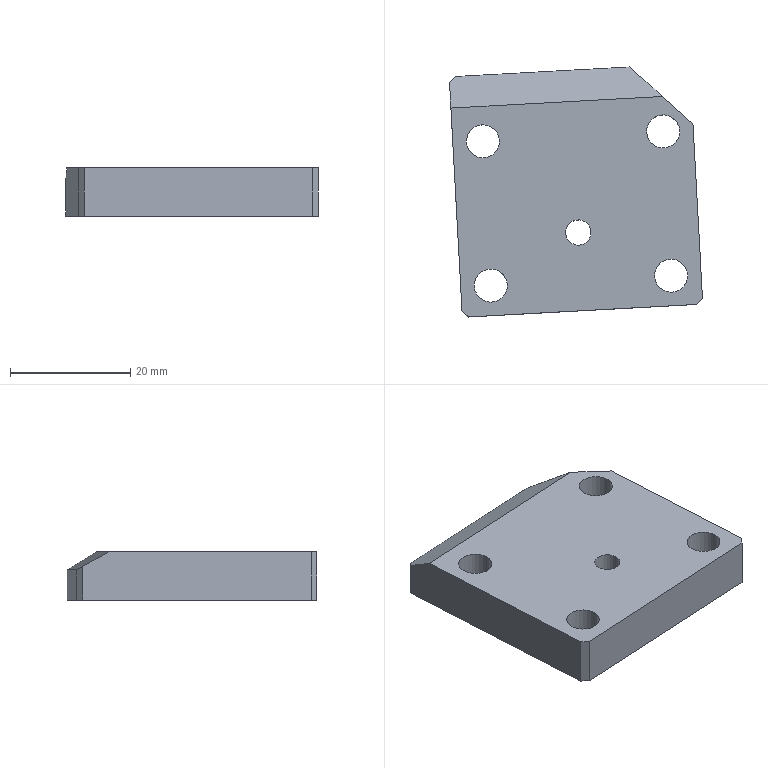Component | SolidWorks | T160418-M01U03-P11A-1 | 1 solid | 24 faces | box 42.02 x 41.53 x 8 mm | volume 10991 mm3 | cylinder 12 | plane 12 | commonest cylinder face diameters 5.5 x8 14 x2 4.2 x2 | material S45C
build123d program:
from build123d import *

# Parameters (mm, degrees)
SKETCH1_W            = 40
SKETCH1_H            = 40
BOSS_EXTRUDE1_DEPTH  = 8
M5_CLEARANCE_HOLE1_D = 5.5
M5_TAPPED_HOLE1_D    = 4.2
CHAMFER1_SIZE        = 10
CHAMFER2_SIZE        = 3
CHAMFER2_SIZE2       = 5.196
CHAMFER3_SIZE        = 1
SKETCH9_R            = 7
CUT_EXTRUDE3_DEPTH   = 2


with BuildPart() as part:
    # Sketch1 → Boss-Extrude1 (new body)
    with BuildSketch(Plane.XY):
        Rectangle(SKETCH1_W, SKETCH1_H)
    extrude(amount=BOSS_EXTRUDE1_DEPTH)

    # M5 Clearance Hole1 (through all)
    with Locations(Plane.XY.offset(8)):
        with Locations((-15, 9), (-15, -15), (15, -15), (15, 9)):
            Hole(M5_CLEARANCE_HOLE1_D / 2)

    # M5 Tapped Hole1 (through all)
    with Locations(Plane.XY.offset(8)):
        with Locations((0, -7)):
            Hole(M5_TAPPED_HOLE1_D / 2)

    # Chamfer1
    chamfer1_edges = [part.edges().sort_by_distance(p)[0] for p in [
        (-20, 20, 4),
    ]]
    chamfer(chamfer1_edges, length=CHAMFER1_SIZE)

    # Chamfer2
    chamfer2_edges = [part.edges().sort_by_distance(p)[0] for p in [
        (5, 20, 0),
    ]]
    chamfer2_side = [part.faces().sort_by_distance(p)[0] for p in [
        (5, 20, 4),
    ]]
    chamfer(chamfer2_edges, length=CHAMFER2_SIZE, length2=CHAMFER2_SIZE2, reference=chamfer2_side[0])

    # Chamfer3
    chamfer3_edges = [part.edges().sort_by_distance(p)[0] for p in [
        (20, -20, 4),
        (-20, -20, 4),
        (20, 20, 5.5),
    ]]
    chamfer(chamfer3_edges, length=CHAMFER3_SIZE)

    # Sketch9 → Cut-Extrude3 (cut)
    with BuildSketch(Plane.XY.offset(8)):
        with Locations((0, -7)):
            Circle(SKETCH9_R)
    extrude(amount=-CUT_EXTRUDE3_DEPTH, mode=Mode.SUBTRACT)


solid = part.part

# Placed as in the assembly
solid = solid.moved(Location((511.102, 149.336, -160.818), (-180, 0, 176.863)))
STEP:
#1=CARTESIAN_POINT('',(20.412,5.619,-6.568));
#2=VERTEX_POINT('',#1);
#3=CARTESIAN_POINT('',(19.862,5.589,-6.568));
#4=VERTEX_POINT('',#3);
#5=CARTESIAN_POINT('',(20.137,5.604,-6.568));
#6=DIRECTION('',(0.,0.,-1.));
#7=DIRECTION('',(-0.9985,-0.05472,0.));
#8=AXIS2_PLACEMENT_3D('',#5,#6,#7);
#9=CIRCLE('',#8,0.2756);
#10=EDGE_CURVE('',#2,#4,#9,.T.);
#11=ORIENTED_EDGE('',*,*,#10,.F.);
#12=CARTESIAN_POINT('',(20.412,5.619,-6.646));
#13=VERTEX_POINT('',#12);
#14=CARTESIAN_POINT('',(20.412,5.619,-6.568));
#15=DIRECTION('',(0.,0.,-1.));
#16=VECTOR('',#15,39.37);
#17=LINE('',#14,#16);
#18=EDGE_CURVE('',#2,#13,#17,.T.);
#19=ORIENTED_EDGE('',*,*,#18,.T.);
#20=CARTESIAN_POINT('',(19.862,5.589,-6.646));
#21=VERTEX_POINT('',#20);
#22=CARTESIAN_POINT('',(20.137,5.604,-6.646));
#23=DIRECTION('',(0.,0.,-1.));
#24=DIRECTION('',(-0.9985,-0.05472,0.));
#25=AXIS2_PLACEMENT_3D('',#22,#23,#24);
#26=CIRCLE('',#25,0.2756);
#27=EDGE_CURVE('',#13,#21,#26,.T.);
#28=ORIENTED_EDGE('',*,*,#27,.T.);
#29=CARTESIAN_POINT('',(19.862,5.589,-6.568));
#30=DIRECTION('',(0.,0.,-1.));
#31=VECTOR('',#30,39.37);
#32=LINE('',#29,#31);
#33=EDGE_CURVE('',#4,#21,#32,.T.);
#34=ORIENTED_EDGE('',*,*,#33,.F.);
#35=EDGE_LOOP('',(#11,#19,#28,#34));
#36=FACE_OUTER_BOUND('',#35,.T.);
#37=CARTESIAN_POINT('',(20.137,5.604,-6.568));
#38=DIRECTION('',(0.,0.,-1.));
#39=DIRECTION('',(-0.9985,-0.05472,0.));
#40=AXIS2_PLACEMENT_3D('',#37,#38,#39);
#41=CYLINDRICAL_SURFACE('',#40,0.2756);
#42=ADVANCED_FACE('',(#36),#41,.F.);
#43=CARTESIAN_POINT('',(20.801,6.271,-6.331));
#44=VERTEX_POINT('',#43);
#45=CARTESIAN_POINT('',(20.584,6.26,-6.331));
#46=VERTEX_POINT('',#45);
#47=CARTESIAN_POINT('',(20.692,6.265,-6.331));
#48=DIRECTION('',(0.,0.,-1.));
#49=DIRECTION('',(-0.9985,-0.05472,0.));
#50=AXIS2_PLACEMENT_3D('',#47,#48,#49);
#51=CIRCLE('',#50,0.1083);
#52=EDGE_CURVE('',#44,#46,#51,.T.);
#53=ORIENTED_EDGE('',*,*,#52,.F.);
#54=CARTESIAN_POINT('',(20.801,6.271,-6.646));
#55=VERTEX_POINT('',#54);
#56=CARTESIAN_POINT('',(20.801,6.271,-6.646));
#57=DIRECTION('',(0.,0.,-1.));
#58=VECTOR('',#57,39.37);
#59=LINE('',#56,#58);
#60=EDGE_CURVE('',#44,#55,#59,.T.);
#61=ORIENTED_EDGE('',*,*,#60,.T.);
#62=CARTESIAN_POINT('',(20.584,6.26,-6.646));
#63=VERTEX_POINT('',#62);
#64=CARTESIAN_POINT('',(20.692,6.265,-6.646));
#65=DIRECTION('',(0.,0.,-1.));
#66=DIRECTION('',(-0.9985,-0.05472,0.));
#67=AXIS2_PLACEMENT_3D('',#64,#65,#66);
#68=CIRCLE('',#67,0.1083);
#69=EDGE_CURVE('',#55,#63,#68,.T.);
#70=ORIENTED_EDGE('',*,*,#69,.T.);
#71=CARTESIAN_POINT('',(20.584,6.26,-6.646));
#72=DIRECTION('',(0.,0.,-1.));
#73=VECTOR('',#72,39.37);
#74=LINE('',#71,#73);
#75=EDGE_CURVE('',#46,#63,#74,.T.);
#76=ORIENTED_EDGE('',*,*,#75,.F.);
#77=EDGE_LOOP('',(#53,#61,#70,#76));
#78=FACE_OUTER_BOUND('',#77,.T.);
#79=CARTESIAN_POINT('',(20.692,6.265,-6.646));
#80=DIRECTION('',(0.,0.,-1.));
#81=DIRECTION('',(-0.9985,-0.05472,0.));
#82=AXIS2_PLACEMENT_3D('',#79,#80,#81);
#83=CYLINDRICAL_SURFACE('',#82,0.1083);
#84=ADVANCED_FACE('',(#78),#83,.F.);
#85=CARTESIAN_POINT('',(20.852,5.328,-6.331));
#86=VERTEX_POINT('',#85);
#87=CARTESIAN_POINT('',(20.636,5.316,-6.331));
#88=VERTEX_POINT('',#87);
#89=CARTESIAN_POINT('',(20.744,5.322,-6.331));
#90=DIRECTION('',(0.,0.,-1.));
#91=DIRECTION('',(-0.9985,-0.05472,0.));
#92=AXIS2_PLACEMENT_3D('',#89,#90,#91);
#93=CIRCLE('',#92,0.1083);
#94=EDGE_CURVE('',#86,#88,#93,.T.);
#95=ORIENTED_EDGE('',*,*,#94,.F.);
#96=CARTESIAN_POINT('',(20.852,5.328,-6.646));
#97=VERTEX_POINT('',#96);
#98=CARTESIAN_POINT('',(20.852,5.328,-6.646));
#99=DIRECTION('',(0.,0.,-1.));
#100=VECTOR('',#99,39.37);
#101=LINE('',#98,#100);
#102=EDGE_CURVE('',#86,#97,#101,.T.);
#103=ORIENTED_EDGE('',*,*,#102,.T.);
#104=CARTESIAN_POINT('',(20.636,5.316,-6.646));
#105=VERTEX_POINT('',#104);
#106=CARTESIAN_POINT('',(20.744,5.322,-6.646));
#107=DIRECTION('',(0.,0.,-1.));
#108=DIRECTION('',(-0.9985,-0.05472,0.));
#109=AXIS2_PLACEMENT_3D('',#106,#107,#108);
#110=CIRCLE('',#109,0.1083);
#111=EDGE_CURVE('',#97,#105,#110,.T.);
#112=ORIENTED_EDGE('',*,*,#111,.T.);
#113=CARTESIAN_POINT('',(20.636,5.316,-6.646));
#114=DIRECTION('',(0.,0.,-1.));
#115=VECTOR('',#114,39.37);
#116=LINE('',#113,#115);
#117=EDGE_CURVE('',#88,#105,#116,.T.);
#118=ORIENTED_EDGE('',*,*,#117,.F.);
#119=EDGE_LOOP('',(#95,#103,#112,#118));
#120=FACE_OUTER_BOUND('',#119,.T.);
#121=CARTESIAN_POINT('',(20.744,5.322,-6.646));
#122=DIRECTION('',(0.,0.,-1.));
#123=DIRECTION('',(-0.9985,-0.05472,0.));
#124=AXIS2_PLACEMENT_3D('',#121,#122,#123);
#125=CYLINDRICAL_SURFACE('',#124,0.1083);
#126=ADVANCED_FACE('',(#120),#125,.F.);
#127=CARTESIAN_POINT('',(19.673,5.263,-6.331));
#128=VERTEX_POINT('',#127);
#129=CARTESIAN_POINT('',(19.457,5.251,-6.331));
#130=VERTEX_POINT('',#129);
#131=CARTESIAN_POINT('',(19.565,5.257,-6.331));
#132=DIRECTION('',(0.,0.,-1.));
#133=DIRECTION('',(-0.9985,-0.05472,0.));
#134=AXIS2_PLACEMENT_3D('',#131,#132,#133);
#135=CIRCLE('',#134,0.1083);
#136=EDGE_CURVE('',#128,#130,#135,.T.);
#137=ORIENTED_EDGE('',*,*,#136,.F.);
#138=CARTESIAN_POINT('',(19.673,5.263,-6.646));
#139=VERTEX_POINT('',#138);
#140=CARTESIAN_POINT('',(19.673,5.263,-6.646));
#141=DIRECTION('',(0.,0.,-1.));
#142=VECTOR('',#141,39.37);
#143=LINE('',#140,#142);
#144=EDGE_CURVE('',#128,#139,#143,.T.);
#145=ORIENTED_EDGE('',*,*,#144,.T.);
#146=CARTESIAN_POINT('',(19.457,5.251,-6.646));
#147=VERTEX_POINT('',#146);
#148=CARTESIAN_POINT('',(19.565,5.257,-6.646));
#149=DIRECTION('',(0.,0.,-1.));
#150=DIRECTION('',(-0.9985,-0.05472,0.));
#151=AXIS2_PLACEMENT_3D('',#148,#149,#150);
#152=CIRCLE('',#151,0.1083);
#153=EDGE_CURVE('',#139,#147,#152,.T.);
#154=ORIENTED_EDGE('',*,*,#153,.T.);
#155=CARTESIAN_POINT('',(19.457,5.251,-6.646));
#156=DIRECTION('',(0.,0.,-1.));
#157=VECTOR('',#156,39.37);
#158=LINE('',#155,#157);
#159=EDGE_CURVE('',#130,#147,#158,.T.);
#160=ORIENTED_EDGE('',*,*,#159,.F.);
#161=EDGE_LOOP('',(#137,#145,#154,#160));
#162=FACE_OUTER_BOUND('',#161,.T.);
#163=CARTESIAN_POINT('',(19.565,5.257,-6.646));
#164=DIRECTION('',(0.,0.,-1.));
#165=DIRECTION('',(-0.9985,-0.05472,0.));
#166=AXIS2_PLACEMENT_3D('',#163,#164,#165);
#167=CYLINDRICAL_SURFACE('',#166,0.1083);
#168=ADVANCED_FACE('',(#162),#167,.F.);
#169=CARTESIAN_POINT('',(19.621,6.207,-6.331));
#170=VERTEX_POINT('',#169);
#171=CARTESIAN_POINT('',(19.405,6.195,-6.331));
#172=VERTEX_POINT('',#171);
#173=CARTESIAN_POINT('',(19.513,6.201,-6.331));
#174=DIRECTION('',(0.,0.,-1.));
#175=DIRECTION('',(-0.9985,-0.05472,0.));
#176=AXIS2_PLACEMENT_3D('',#173,#174,#175);
#177=CIRCLE('',#176,0.1083);
#178=EDGE_CURVE('',#170,#172,#177,.T.);
#179=ORIENTED_EDGE('',*,*,#178,.F.);
#180=CARTESIAN_POINT('',(19.621,6.207,-6.646));
#181=VERTEX_POINT('',#180);
#182=CARTESIAN_POINT('',(19.621,6.207,-6.646));
#183=DIRECTION('',(0.,0.,-1.));
#184=VECTOR('',#183,39.37);
#185=LINE('',#182,#184);
#186=EDGE_CURVE('',#170,#181,#185,.T.);
#187=ORIENTED_EDGE('',*,*,#186,.T.);
#188=CARTESIAN_POINT('',(19.405,6.195,-6.646));
#189=VERTEX_POINT('',#188);
#190=CARTESIAN_POINT('',(19.513,6.201,-6.646));
#191=DIRECTION('',(0.,0.,-1.));
#192=DIRECTION('',(-0.9985,-0.05472,0.));
#193=AXIS2_PLACEMENT_3D('',#190,#191,#192);
#194=CIRCLE('',#193,0.1083);
#195=EDGE_CURVE('',#181,#189,#194,.T.);
#196=ORIENTED_EDGE('',*,*,#195,.T.);
#197=CARTESIAN_POINT('',(19.405,6.195,-6.646));
#198=DIRECTION('',(0.,0.,-1.));
#199=VECTOR('',#198,39.37);
#200=LINE('',#197,#199);
#201=EDGE_CURVE('',#172,#189,#200,.T.);
#202=ORIENTED_EDGE('',*,*,#201,.F.);
#203=EDGE_LOOP('',(#179,#187,#196,#202));
#204=FACE_OUTER_BOUND('',#203,.T.);
#205=CARTESIAN_POINT('',(19.513,6.201,-6.646));
#206=DIRECTION('',(0.,0.,-1.));
#207=DIRECTION('',(-0.9985,-0.05472,0.));
#208=AXIS2_PLACEMENT_3D('',#205,#206,#207);
#209=CYLINDRICAL_SURFACE('',#208,0.1083);
#210=ADVANCED_FACE('',(#204),#209,.F.);
#211=CARTESIAN_POINT('',(20.22,5.609,-6.331));
#212=VERTEX_POINT('',#211);
#213=CARTESIAN_POINT('',(20.055,5.6,-6.331));
#214=VERTEX_POINT('',#213);
#215=CARTESIAN_POINT('',(20.137,5.604,-6.331));
#216=DIRECTION('',(0.,0.,-1.));
#217=DIRECTION('',(-0.9985,-0.05472,0.));
#218=AXIS2_PLACEMENT_3D('',#215,#216,#217);
#219=CIRCLE('',#218,0.08268);
#220=EDGE_CURVE('',#212,#214,#219,.T.);
#221=ORIENTED_EDGE('',*,*,#220,.F.);
#222=CARTESIAN_POINT('',(20.22,5.609,-6.568));
#223=VERTEX_POINT('',#222);
#224=CARTESIAN_POINT('',(20.22,5.609,-6.646));
#225=DIRECTION('',(0.,0.,-1.));
#226=VECTOR('',#225,39.37);
#227=LINE('',#224,#226);
#228=EDGE_CURVE('',#212,#223,#227,.T.);
#229=ORIENTED_EDGE('',*,*,#228,.T.);
#230=CARTESIAN_POINT('',(20.055,5.6,-6.568));
#231=VERTEX_POINT('',#230);
#232=CARTESIAN_POINT('',(20.137,5.604,-6.568));
#233=DIRECTION('',(-0.,-0.,1.));
#234=DIRECTION('',(-0.9985,-0.05472,0.));
#235=AXIS2_PLACEMENT_3D('',#232,#233,#234);
#236=CIRCLE('',#235,0.08268);
#237=EDGE_CURVE('',#231,#223,#236,.T.);
#238=ORIENTED_EDGE('',*,*,#237,.F.);
#239=CARTESIAN_POINT('',(20.055,5.6,-6.646));
#240=DIRECTION('',(0.,0.,-1.));
#241=VECTOR('',#240,39.37);
#242=LINE('',#239,#241);
#243=EDGE_CURVE('',#214,#231,#242,.T.);
#244=ORIENTED_EDGE('',*,*,#243,.F.);
#245=EDGE_LOOP('',(#221,#229,#238,#244));
#246=FACE_OUTER_BOUND('',#245,.T.);
#247=CARTESIAN_POINT('',(20.137,5.604,-6.646));
#248=DIRECTION('',(0.,0.,-1.));
#249=DIRECTION('',(-0.9985,-0.05472,0.));
#250=AXIS2_PLACEMENT_3D('',#247,#248,#249);
#251=CYLINDRICAL_SURFACE('',#250,0.08268);
#252=ADVANCED_FACE('',(#246),#251,.F.);
#253=ORIENTED_EDGE('',*,*,#228,.F.);
#254=CARTESIAN_POINT('',(20.137,5.604,-6.331));
#255=DIRECTION('',(0.,0.,-1.));
#256=DIRECTION('',(-0.9985,-0.05472,0.));
#257=AXIS2_PLACEMENT_3D('',#254,#255,#256);
#258=CIRCLE('',#257,0.08268);
#259=EDGE_CURVE('',#214,#212,#258,.T.);
#260=ORIENTED_EDGE('',*,*,#259,.F.);
#261=ORIENTED_EDGE('',*,*,#243,.T.);
#262=CARTESIAN_POINT('',(20.137,5.604,-6.568));
#263=DIRECTION('',(-0.,-0.,1.));
#264=DIRECTION('',(-0.9985,-0.05472,0.));
#265=AXIS2_PLACEMENT_3D('',#262,#263,#264);
#266=CIRCLE('',#265,0.08268);
#267=EDGE_CURVE('',#223,#231,#266,.T.);
#268=ORIENTED_EDGE('',*,*,#267,.F.);
#269=EDGE_LOOP('',(#253,#260,#261,#268));
#270=FACE_OUTER_BOUND('',#269,.T.);
#271=CARTESIAN_POINT('',(20.137,5.604,-6.646));
#272=DIRECTION('',(0.,0.,-1.));
#273=DIRECTION('',(-0.9985,-0.05472,0.));
#274=AXIS2_PLACEMENT_3D('',#271,#272,#273);
#275=CYLINDRICAL_SURFACE('',#274,0.08268);
#276=ADVANCED_FACE('',(#270),#275,.F.);
#277=CARTESIAN_POINT('',(19.304,6.418,-6.331));
#278=VERTEX_POINT('',#277);
#279=CARTESIAN_POINT('',(19.295,6.583,-6.427));
#280=VERTEX_POINT('',#279);
#281=CARTESIAN_POINT('',(19.293,6.623,-6.45));
#282=DIRECTION('',(-0.04739,0.8647,-0.5));
#283=VECTOR('',#282,39.37);
#284=LINE('',#281,#283);
#285=EDGE_CURVE('',#278,#280,#284,.T.);
#286=ORIENTED_EDGE('',*,*,#285,.T.);
#287=CARTESIAN_POINT('',(19.295,6.583,-6.646));
#288=VERTEX_POINT('',#287);
#289=CARTESIAN_POINT('',(19.295,6.583,-6.646));
#290=DIRECTION('',(0.,0.,-1.));
#291=VECTOR('',#290,39.37);
#292=LINE('',#289,#291);
#293=EDGE_CURVE('',#280,#288,#292,.T.);
#294=ORIENTED_EDGE('',*,*,#293,.T.);
#295=CARTESIAN_POINT('',(19.377,5.089,-6.646));
#296=VERTEX_POINT('',#295);
#297=CARTESIAN_POINT('',(19.293,6.623,-6.646));
#298=DIRECTION('',(-0.05472,0.9985,0.));
#299=VECTOR('',#298,39.37);
#300=LINE('',#297,#299);
#301=EDGE_CURVE('',#296,#288,#300,.T.);
#302=ORIENTED_EDGE('',*,*,#301,.F.);
#303=CARTESIAN_POINT('',(19.377,5.089,-6.331));
#304=VERTEX_POINT('',#303);
#305=CARTESIAN_POINT('',(19.377,5.089,-6.646));
#306=DIRECTION('',(-0.,-0.,1.));
#307=VECTOR('',#306,39.37);
#308=LINE('',#305,#307);
#309=EDGE_CURVE('',#296,#304,#308,.T.);
#310=ORIENTED_EDGE('',*,*,#309,.T.);
#311=CARTESIAN_POINT('',(19.293,6.623,-6.331));
#312=DIRECTION('',(-0.05472,0.9985,0.));
#313=VECTOR('',#312,39.37);
#314=LINE('',#311,#313);
#315=EDGE_CURVE('',#304,#278,#314,.T.);
#316=ORIENTED_EDGE('',*,*,#315,.T.);
#317=EDGE_LOOP('',(#286,#294,#302,#310,#316));
#318=FACE_OUTER_BOUND('',#317,.T.);
#319=CARTESIAN_POINT('',(19.293,6.623,-6.646));
#320=DIRECTION('',(0.9985,0.05472,0.));
#321=DIRECTION('',(0.05472,-0.9985,-0.));
#322=AXIS2_PLACEMENT_3D('',#319,#320,#321);
#323=PLANE('',#322);
#324=ADVANCED_FACE('',(#318),#323,.F.);
#325=CARTESIAN_POINT('',(19.332,6.625,-6.646));
#326=VERTEX_POINT('',#325);
#327=CARTESIAN_POINT('',(20.472,6.687,-6.646));
#328=VERTEX_POINT('',#327);
#329=CARTESIAN_POINT('',(20.865,6.709,-6.646));
#330=DIRECTION('',(0.9985,0.05472,0.));
#331=VECTOR('',#330,39.37);
#332=LINE('',#329,#331);
#333=EDGE_CURVE('',#326,#328,#332,.T.);
#334=ORIENTED_EDGE('',*,*,#333,.F.);
#335=CARTESIAN_POINT('',(19.332,6.625,-6.45));
#336=VERTEX_POINT('',#335);
#337=CARTESIAN_POINT('',(19.332,6.625,-6.646));
#338=DIRECTION('',(-0.,-0.,1.));
#339=VECTOR('',#338,39.37);
#340=LINE('',#337,#339);
#341=EDGE_CURVE('',#326,#336,#340,.T.);
#342=ORIENTED_EDGE('',*,*,#341,.T.);
#343=CARTESIAN_POINT('',(20.472,6.687,-6.45));
#344=VERTEX_POINT('',#343);
#345=CARTESIAN_POINT('',(20.865,6.709,-6.45));
#346=DIRECTION('',(0.9985,0.05472,0.));
#347=VECTOR('',#346,39.37);
#348=LINE('',#345,#347);
#349=EDGE_CURVE('',#336,#344,#348,.T.);
#350=ORIENTED_EDGE('',*,*,#349,.T.);
#351=CARTESIAN_POINT('',(20.472,6.687,-6.646));
#352=DIRECTION('',(0.,0.,-1.));
#353=VECTOR('',#352,39.37);
#354=LINE('',#351,#353);
#355=EDGE_CURVE('',#344,#328,#354,.T.);
#356=ORIENTED_EDGE('',*,*,#355,.T.);
#357=EDGE_LOOP('',(#334,#342,#350,#356));
#358=FACE_OUTER_BOUND('',#357,.T.);
#359=CARTESIAN_POINT('',(20.865,6.709,-6.646));
#360=DIRECTION('',(0.05472,-0.9985,-0.));
#361=DIRECTION('',(-0.,-0.,1.));
#362=AXIS2_PLACEMENT_3D('',#359,#360,#361);
#363=PLANE('',#362);
#364=ADVANCED_FACE('',(#358),#363,.F.);
#365=CARTESIAN_POINT('',(20.887,6.316,-6.331));
#366=VERTEX_POINT('',#365);
#367=CARTESIAN_POINT('',(20.949,5.176,-6.331));
#368=VERTEX_POINT('',#367);
#369=CARTESIAN_POINT('',(20.865,6.709,-6.331));
#370=DIRECTION('',(0.05472,-0.9985,-0.));
#371=VECTOR('',#370,39.37);
#372=LINE('',#369,#371);
#373=EDGE_CURVE('',#366,#368,#372,.T.);
#374=ORIENTED_EDGE('',*,*,#373,.T.);
#375=CARTESIAN_POINT('',(20.949,5.176,-6.646));
#376=VERTEX_POINT('',#375);
#377=CARTESIAN_POINT('',(20.949,5.176,-6.646));
#378=DIRECTION('',(0.,0.,-1.));
#379=VECTOR('',#378,39.37);
#380=LINE('',#377,#379);
#381=EDGE_CURVE('',#368,#376,#380,.T.);
#382=ORIENTED_EDGE('',*,*,#381,.T.);
#383=CARTESIAN_POINT('',(20.887,6.316,-6.646));
#384=VERTEX_POINT('',#383);
#385=CARTESIAN_POINT('',(20.865,6.709,-6.646));
#386=DIRECTION('',(0.05472,-0.9985,-0.));
#387=VECTOR('',#386,39.37);
#388=LINE('',#385,#387);
#389=EDGE_CURVE('',#384,#376,#388,.T.);
#390=ORIENTED_EDGE('',*,*,#389,.F.);
#391=CARTESIAN_POINT('',(20.887,6.316,-6.646));
#392=DIRECTION('',(-0.,-0.,1.));
#393=VECTOR('',#392,39.37);
#394=LINE('',#391,#393);
#395=EDGE_CURVE('',#384,#366,#394,.T.);
#396=ORIENTED_EDGE('',*,*,#395,.T.);
#397=EDGE_LOOP('',(#374,#382,#390,#396));
#398=FACE_OUTER_BOUND('',#397,.T.);
#399=CARTESIAN_POINT('',(20.865,6.709,-6.646));
#400=DIRECTION('',(-0.9985,-0.05472,-0.));
#401=DIRECTION('',(-0.05472,0.9985,0.));
#402=AXIS2_PLACEMENT_3D('',#399,#400,#401);
#403=PLANE('',#402);
#404=ADVANCED_FACE('',(#398),#403,.F.);
#405=CARTESIAN_POINT('',(20.912,5.134,-6.646));
#406=VERTEX_POINT('',#405);
#407=CARTESIAN_POINT('',(19.418,5.052,-6.646));
#408=VERTEX_POINT('',#407);
#409=CARTESIAN_POINT('',(20.951,5.136,-6.646));
#410=DIRECTION('',(-0.9985,-0.05472,-0.));
#411=VECTOR('',#410,39.37);
#412=LINE('',#409,#411);
#413=EDGE_CURVE('',#406,#408,#412,.T.);
#414=ORIENTED_EDGE('',*,*,#413,.F.);
#415=CARTESIAN_POINT('',(20.912,5.134,-6.331));
#416=VERTEX_POINT('',#415);
#417=CARTESIAN_POINT('',(20.912,5.134,-6.646));
#418=DIRECTION('',(-0.,-0.,1.));
#419=VECTOR('',#418,39.37);
#420=LINE('',#417,#419);
#421=EDGE_CURVE('',#406,#416,#420,.T.);
#422=ORIENTED_EDGE('',*,*,#421,.T.);
#423=CARTESIAN_POINT('',(19.418,5.052,-6.331));
#424=VERTEX_POINT('',#423);
#425=CARTESIAN_POINT('',(20.951,5.136,-6.331));
#426=DIRECTION('',(-0.9985,-0.05472,-0.));
#427=VECTOR('',#426,39.37);
#428=LINE('',#425,#427);
#429=EDGE_CURVE('',#416,#424,#428,.T.);
#430=ORIENTED_EDGE('',*,*,#429,.T.);
#431=CARTESIAN_POINT('',(19.418,5.052,-6.646));
#432=DIRECTION('',(0.,0.,-1.));
#433=VECTOR('',#432,39.37);
#434=LINE('',#431,#433);
#435=EDGE_CURVE('',#424,#408,#434,.T.);
#436=ORIENTED_EDGE('',*,*,#435,.T.);
#437=EDGE_LOOP('',(#414,#422,#430,#436));
#438=FACE_OUTER_BOUND('',#437,.T.);
#439=CARTESIAN_POINT('',(20.951,5.136,-6.646));
#440=DIRECTION('',(-0.05472,0.9985,0.));
#441=DIRECTION('',(0.,0.,-1.));
#442=AXIS2_PLACEMENT_3D('',#439,#440,#441);
#443=PLANE('',#442);
#444=ADVANCED_FACE('',(#438),#443,.F.);
#445=CARTESIAN_POINT('',(20.137,5.604,-6.646));
#446=DIRECTION('',(0.,0.,-1.));
#447=DIRECTION('',(-0.9985,-0.05472,0.));
#448=AXIS2_PLACEMENT_3D('',#445,#446,#447);
#449=CIRCLE('',#448,0.2756);
#450=EDGE_CURVE('',#21,#13,#449,.T.);
#451=ORIENTED_EDGE('',*,*,#450,.F.);
#452=ORIENTED_EDGE('',*,*,#27,.F.);
#453=EDGE_LOOP('',(#451,#452));
#454=FACE_BOUND('',#453,.T.);
#455=CARTESIAN_POINT('',(20.692,6.265,-6.646));
#456=DIRECTION('',(0.,0.,-1.));
#457=DIRECTION('',(-0.9985,-0.05472,0.));
#458=AXIS2_PLACEMENT_3D('',#455,#456,#457);
#459=CIRCLE('',#458,0.1083);
#460=EDGE_CURVE('',#63,#55,#459,.T.);
#461=ORIENTED_EDGE('',*,*,#460,.F.);
#462=ORIENTED_EDGE('',*,*,#69,.F.);
#463=EDGE_LOOP('',(#461,#462));
#464=FACE_BOUND('',#463,.T.);
#465=CARTESIAN_POINT('',(20.744,5.322,-6.646));
#466=DIRECTION('',(0.,0.,-1.));
#467=DIRECTION('',(-0.9985,-0.05472,0.));
#468=AXIS2_PLACEMENT_3D('',#465,#466,#467);
#469=CIRCLE('',#468,0.1083);
#470=EDGE_CURVE('',#105,#97,#469,.T.);
#471=ORIENTED_EDGE('',*,*,#470,.F.);
#472=ORIENTED_EDGE('',*,*,#111,.F.);
#473=EDGE_LOOP('',(#471,#472));
#474=FACE_BOUND('',#473,.T.);
#475=CARTESIAN_POINT('',(19.565,5.257,-6.646));
#476=DIRECTION('',(0.,0.,-1.));
#477=DIRECTION('',(-0.9985,-0.05472,0.));
#478=AXIS2_PLACEMENT_3D('',#475,#476,#477);
#479=CIRCLE('',#478,0.1083);
#480=EDGE_CURVE('',#147,#139,#479,.T.);
#481=ORIENTED_EDGE('',*,*,#480,.F.);
#482=ORIENTED_EDGE('',*,*,#153,.F.);
#483=EDGE_LOOP('',(#481,#482));
#484=FACE_BOUND('',#483,.T.);
#485=CARTESIAN_POINT('',(19.513,6.201,-6.646));
#486=DIRECTION('',(0.,0.,-1.));
#487=DIRECTION('',(-0.9985,-0.05472,0.));
#488=AXIS2_PLACEMENT_3D('',#485,#486,#487);
#489=CIRCLE('',#488,0.1083);
#490=EDGE_CURVE('',#189,#181,#489,.T.);
#491=ORIENTED_EDGE('',*,*,#490,.F.);
#492=ORIENTED_EDGE('',*,*,#195,.F.);
#493=EDGE_LOOP('',(#491,#492));
#494=FACE_BOUND('',#493,.T.);
#495=ORIENTED_EDGE('',*,*,#301,.T.);
#496=CARTESIAN_POINT('',(18.57,5.775,-6.646));
#497=DIRECTION('',(0.6674,0.7447,0.));
#498=VECTOR('',#497,39.37);
#499=LINE('',#496,#498);
#500=EDGE_CURVE('',#288,#326,#499,.T.);
#501=ORIENTED_EDGE('',*,*,#500,.T.);
#502=ORIENTED_EDGE('',*,*,#333,.T.);
#503=CARTESIAN_POINT('',(20.679,6.501,-6.646));
#504=DIRECTION('',(0.7447,-0.6674,0.));
#505=VECTOR('',#504,39.37);
#506=LINE('',#503,#505);
#507=EDGE_CURVE('',#328,#384,#506,.T.);
#508=ORIENTED_EDGE('',*,*,#507,.T.);
#509=ORIENTED_EDGE('',*,*,#389,.T.);
#510=CARTESIAN_POINT('',(20.188,4.326,-6.646));
#511=DIRECTION('',(-0.6674,-0.7447,-0.));
#512=VECTOR('',#511,39.37);
#513=LINE('',#510,#512);
#514=EDGE_CURVE('',#376,#406,#513,.T.);
#515=ORIENTED_EDGE('',*,*,#514,.T.);
#516=ORIENTED_EDGE('',*,*,#413,.T.);
#517=CARTESIAN_POINT('',(19.398,5.071,-6.646));
#518=DIRECTION('',(-0.7447,0.6674,-0.));
#519=VECTOR('',#518,39.37);
#520=LINE('',#517,#519);
#521=EDGE_CURVE('',#408,#296,#520,.T.);
#522=ORIENTED_EDGE('',*,*,#521,.T.);
#523=EDGE_LOOP('',(#495,#501,#502,#508,#509,#515,#516,#522));
#524=FACE_OUTER_BOUND('',#523,.T.);
#525=CARTESIAN_POINT('',(19.379,5.05,-6.646));
#526=DIRECTION('',(0.,0.,-1.));
#527=DIRECTION('',(-0.9985,-0.05472,-0.));
#528=AXIS2_PLACEMENT_3D('',#525,#526,#527);
#529=PLANE('',#528);
#530=ADVANCED_FACE('',(#454,#464,#474,#484,#494,#524),#529,.T.);
#531=ORIENTED_EDGE('',*,*,#259,.T.);
#532=ORIENTED_EDGE('',*,*,#220,.T.);
#533=EDGE_LOOP('',(#531,#532));
#534=FACE_BOUND('',#533,.T.);
#535=CARTESIAN_POINT('',(20.692,6.265,-6.331));
#536=DIRECTION('',(0.,0.,-1.));
#537=DIRECTION('',(-0.9985,-0.05472,0.));
#538=AXIS2_PLACEMENT_3D('',#535,#536,#537);
#539=CIRCLE('',#538,0.1083);
#540=EDGE_CURVE('',#46,#44,#539,.T.);
#541=ORIENTED_EDGE('',*,*,#540,.T.);
#542=ORIENTED_EDGE('',*,*,#52,.T.);
#543=EDGE_LOOP('',(#541,#542));
#544=FACE_BOUND('',#543,.T.);
#545=CARTESIAN_POINT('',(20.744,5.322,-6.331));
#546=DIRECTION('',(0.,0.,-1.));
#547=DIRECTION('',(-0.9985,-0.05472,0.));
#548=AXIS2_PLACEMENT_3D('',#545,#546,#547);
#549=CIRCLE('',#548,0.1083);
#550=EDGE_CURVE('',#88,#86,#549,.T.);
#551=ORIENTED_EDGE('',*,*,#550,.T.);
#552=ORIENTED_EDGE('',*,*,#94,.T.);
#553=EDGE_LOOP('',(#551,#552));
#554=FACE_BOUND('',#553,.T.);
#555=CARTESIAN_POINT('',(19.565,5.257,-6.331));
#556=DIRECTION('',(0.,0.,-1.));
#557=DIRECTION('',(-0.9985,-0.05472,0.));
#558=AXIS2_PLACEMENT_3D('',#555,#556,#557);
#559=CIRCLE('',#558,0.1083);
#560=EDGE_CURVE('',#130,#128,#559,.T.);
#561=ORIENTED_EDGE('',*,*,#560,.T.);
#562=ORIENTED_EDGE('',*,*,#136,.T.);
#563=EDGE_LOOP('',(#561,#562));
#564=FACE_BOUND('',#563,.T.);
#565=CARTESIAN_POINT('',(19.513,6.201,-6.331));
#566=DIRECTION('',(0.,0.,-1.));
#567=DIRECTION('',(-0.9985,-0.05472,0.));
#568=AXIS2_PLACEMENT_3D('',#565,#566,#567);
#569=CIRCLE('',#568,0.1083);
#570=EDGE_CURVE('',#172,#170,#569,.T.);
#571=ORIENTED_EDGE('',*,*,#570,.T.);
#572=ORIENTED_EDGE('',*,*,#178,.T.);
#573=EDGE_LOOP('',(#571,#572));
#574=FACE_BOUND('',#573,.T.);
#575=ORIENTED_EDGE('',*,*,#429,.F.);
#576=CARTESIAN_POINT('',(20.912,5.134,-6.331));
#577=DIRECTION('',(0.6674,0.7447,0.));
#578=VECTOR('',#577,39.37);
#579=LINE('',#576,#578);
#580=EDGE_CURVE('',#416,#368,#579,.T.);
#581=ORIENTED_EDGE('',*,*,#580,.T.);
#582=ORIENTED_EDGE('',*,*,#373,.F.);
#583=CARTESIAN_POINT('',(20.688,6.494,-6.331));
#584=VERTEX_POINT('',#583);
#585=CARTESIAN_POINT('',(20.887,6.316,-6.331));
#586=DIRECTION('',(-0.7447,0.6674,-0.));
#587=VECTOR('',#586,39.37);
#588=LINE('',#585,#587);
#589=EDGE_CURVE('',#366,#584,#588,.T.);
#590=ORIENTED_EDGE('',*,*,#589,.T.);
#591=CARTESIAN_POINT('',(19.304,6.418,-6.331));
#592=DIRECTION('',(-0.9985,-0.05472,-0.));
#593=VECTOR('',#592,39.37);
#594=LINE('',#591,#593);
#595=EDGE_CURVE('',#584,#278,#594,.T.);
#596=ORIENTED_EDGE('',*,*,#595,.T.);
#597=ORIENTED_EDGE('',*,*,#315,.F.);
#598=CARTESIAN_POINT('',(19.377,5.089,-6.331));
#599=DIRECTION('',(0.7447,-0.6674,0.));
#600=VECTOR('',#599,39.37);
#601=LINE('',#598,#600);
#602=EDGE_CURVE('',#304,#424,#601,.T.);
#603=ORIENTED_EDGE('',*,*,#602,.T.);
#604=EDGE_LOOP('',(#575,#581,#582,#590,#596,#597,#603));
#605=FACE_OUTER_BOUND('',#604,.T.);
#606=CARTESIAN_POINT('',(19.379,5.05,-6.331));
#607=DIRECTION('',(0.,0.,-1.));
#608=DIRECTION('',(-0.9985,-0.05472,-0.));
#609=AXIS2_PLACEMENT_3D('',#606,#607,#608);
#610=PLANE('',#609);
#611=ADVANCED_FACE('',(#534,#544,#554,#564,#574,#605),#610,.F.);
#612=ORIENTED_EDGE('',*,*,#186,.F.);
#613=ORIENTED_EDGE('',*,*,#570,.F.);
#614=ORIENTED_EDGE('',*,*,#201,.T.);
#615=ORIENTED_EDGE('',*,*,#490,.T.);
#616=EDGE_LOOP('',(#612,#613,#614,#615));
#617=FACE_OUTER_BOUND('',#616,.T.);
#618=CARTESIAN_POINT('',(19.513,6.201,-6.646));
#619=DIRECTION('',(0.,0.,-1.));
#620=DIRECTION('',(-0.9985,-0.05472,0.));
#621=AXIS2_PLACEMENT_3D('',#618,#619,#620);
#622=CYLINDRICAL_SURFACE('',#621,0.1083);
#623=ADVANCED_FACE('',(#617),#622,.F.);
#624=ORIENTED_EDGE('',*,*,#144,.F.);
#625=ORIENTED_EDGE('',*,*,#560,.F.);
#626=ORIENTED_EDGE('',*,*,#159,.T.);
#627=ORIENTED_EDGE('',*,*,#480,.T.);
#628=EDGE_LOOP('',(#624,#625,#626,#627));
#629=FACE_OUTER_BOUND('',#628,.T.);
#630=CARTESIAN_POINT('',(19.565,5.257,-6.646));
#631=DIRECTION('',(0.,0.,-1.));
#632=DIRECTION('',(-0.9985,-0.05472,0.));
#633=AXIS2_PLACEMENT_3D('',#630,#631,#632);
#634=CYLINDRICAL_SURFACE('',#633,0.1083);
#635=ADVANCED_FACE('',(#629),#634,.F.);
#636=ORIENTED_EDGE('',*,*,#102,.F.);
#637=ORIENTED_EDGE('',*,*,#550,.F.);
#638=ORIENTED_EDGE('',*,*,#117,.T.);
#639=ORIENTED_EDGE('',*,*,#470,.T.);
#640=EDGE_LOOP('',(#636,#637,#638,#639));
#641=FACE_OUTER_BOUND('',#640,.T.);
#642=CARTESIAN_POINT('',(20.744,5.322,-6.646));
#643=DIRECTION('',(0.,0.,-1.));
#644=DIRECTION('',(-0.9985,-0.05472,0.));
#645=AXIS2_PLACEMENT_3D('',#642,#643,#644);
#646=CYLINDRICAL_SURFACE('',#645,0.1083);
#647=ADVANCED_FACE('',(#641),#646,.F.);
#648=ORIENTED_EDGE('',*,*,#60,.F.);
#649=ORIENTED_EDGE('',*,*,#540,.F.);
#650=ORIENTED_EDGE('',*,*,#75,.T.);
#651=ORIENTED_EDGE('',*,*,#460,.T.);
#652=EDGE_LOOP('',(#648,#649,#650,#651));
#653=FACE_OUTER_BOUND('',#652,.T.);
#654=CARTESIAN_POINT('',(20.692,6.265,-6.646));
#655=DIRECTION('',(0.,0.,-1.));
#656=DIRECTION('',(-0.9985,-0.05472,0.));
#657=AXIS2_PLACEMENT_3D('',#654,#655,#656);
#658=CYLINDRICAL_SURFACE('',#657,0.1083);
#659=ADVANCED_FACE('',(#653),#658,.F.);
#660=ORIENTED_EDGE('',*,*,#355,.F.);
#661=CARTESIAN_POINT('',(20.776,6.415,-6.283));
#662=DIRECTION('',(0.6895,-0.6179,0.378));
#663=VECTOR('',#662,39.37);
#664=LINE('',#661,#663);
#665=EDGE_CURVE('',#344,#584,#664,.T.);
#666=ORIENTED_EDGE('',*,*,#665,.T.);
#667=ORIENTED_EDGE('',*,*,#589,.F.);
#668=ORIENTED_EDGE('',*,*,#395,.F.);
#669=ORIENTED_EDGE('',*,*,#507,.F.);
#670=EDGE_LOOP('',(#660,#666,#667,#668,#669));
#671=FACE_OUTER_BOUND('',#670,.T.);
#672=CARTESIAN_POINT('',(20.887,6.316,-6.646));
#673=DIRECTION('',(-0.6674,-0.7447,-0.));
#674=DIRECTION('',(-0.7447,0.6674,-0.));
#675=AXIS2_PLACEMENT_3D('',#672,#673,#674);
#676=PLANE('',#675);
#677=ADVANCED_FACE('',(#671),#676,.F.);
#678=ORIENTED_EDGE('',*,*,#349,.F.);
#679=CARTESIAN_POINT('',(19.953,7.318,-6.829));
#680=DIRECTION('',(-0.6179,-0.6895,0.378));
#681=VECTOR('',#680,39.37);
#682=LINE('',#679,#681);
#683=EDGE_CURVE('',#336,#280,#682,.T.);
#684=ORIENTED_EDGE('',*,*,#683,.T.);
#685=ORIENTED_EDGE('',*,*,#285,.F.);
#686=ORIENTED_EDGE('',*,*,#595,.F.);
#687=ORIENTED_EDGE('',*,*,#665,.F.);
#688=EDGE_LOOP('',(#678,#684,#685,#686,#687));
#689=FACE_OUTER_BOUND('',#688,.T.);
#690=CARTESIAN_POINT('',(20.865,6.709,-6.45));
#691=DIRECTION('',(0.02736,-0.4993,-0.866));
#692=DIRECTION('',(0.04739,-0.8647,0.5));
#693=AXIS2_PLACEMENT_3D('',#690,#691,#692);
#694=PLANE('',#693);
#695=ADVANCED_FACE('',(#689),#694,.F.);
#696=ORIENTED_EDGE('',*,*,#500,.F.);
#697=ORIENTED_EDGE('',*,*,#293,.F.);
#698=ORIENTED_EDGE('',*,*,#683,.F.);
#699=ORIENTED_EDGE('',*,*,#341,.F.);
#700=EDGE_LOOP('',(#696,#697,#698,#699));
#701=FACE_OUTER_BOUND('',#700,.T.);
#702=CARTESIAN_POINT('',(19.332,6.625,-6.646));
#703=DIRECTION('',(0.7447,-0.6674,0.));
#704=DIRECTION('',(-0.6674,-0.7447,-0.));
#705=AXIS2_PLACEMENT_3D('',#702,#703,#704);
#706=PLANE('',#705);
#707=ADVANCED_FACE('',(#701),#706,.F.);
#708=ORIENTED_EDGE('',*,*,#514,.F.);
#709=ORIENTED_EDGE('',*,*,#381,.F.);
#710=ORIENTED_EDGE('',*,*,#580,.F.);
#711=ORIENTED_EDGE('',*,*,#421,.F.);
#712=EDGE_LOOP('',(#708,#709,#710,#711));
#713=FACE_OUTER_BOUND('',#712,.T.);
#714=CARTESIAN_POINT('',(20.912,5.134,-6.646));
#715=DIRECTION('',(-0.7447,0.6674,-0.));
#716=DIRECTION('',(0.6674,0.7447,0.));
#717=AXIS2_PLACEMENT_3D('',#714,#715,#716);
#718=PLANE('',#717);
#719=ADVANCED_FACE('',(#713),#718,.F.);
#720=ORIENTED_EDGE('',*,*,#521,.F.);
#721=ORIENTED_EDGE('',*,*,#435,.F.);
#722=ORIENTED_EDGE('',*,*,#602,.F.);
#723=ORIENTED_EDGE('',*,*,#309,.F.);
#724=EDGE_LOOP('',(#720,#721,#722,#723));
#725=FACE_OUTER_BOUND('',#724,.T.);
#726=CARTESIAN_POINT('',(19.377,5.089,-6.646));
#727=DIRECTION('',(0.6674,0.7447,0.));
#728=DIRECTION('',(0.7447,-0.6674,0.));
#729=AXIS2_PLACEMENT_3D('',#726,#727,#728);
#730=PLANE('',#729);
#731=ADVANCED_FACE('',(#725),#730,.F.);
#732=CARTESIAN_POINT('',(20.137,5.604,-6.568));
#733=DIRECTION('',(0.,0.,-1.));
#734=DIRECTION('',(-0.9985,-0.05472,0.));
#735=AXIS2_PLACEMENT_3D('',#732,#733,#734);
#736=CIRCLE('',#735,0.2756);
#737=EDGE_CURVE('',#4,#2,#736,.T.);
#738=ORIENTED_EDGE('',*,*,#737,.T.);
#739=ORIENTED_EDGE('',*,*,#10,.T.);
#740=EDGE_LOOP('',(#738,#739));
#741=FACE_OUTER_BOUND('',#740,.T.);
#742=ORIENTED_EDGE('',*,*,#237,.T.);
#743=ORIENTED_EDGE('',*,*,#267,.T.);
#744=EDGE_LOOP('',(#742,#743));
#745=FACE_BOUND('',#744,.T.);
#746=CARTESIAN_POINT('',(20.137,5.604,-6.568));
#747=DIRECTION('',(0.,0.,-1.));
#748=DIRECTION('',(-0.9985,-0.05472,-0.));
#749=AXIS2_PLACEMENT_3D('',#746,#747,#748);
#750=PLANE('',#749);
#751=ADVANCED_FACE('',(#741,#745),#750,.T.);
#752=ORIENTED_EDGE('',*,*,#18,.F.);
#753=ORIENTED_EDGE('',*,*,#737,.F.);
#754=ORIENTED_EDGE('',*,*,#33,.T.);
#755=ORIENTED_EDGE('',*,*,#450,.T.);
#756=EDGE_LOOP('',(#752,#753,#754,#755));
#757=FACE_OUTER_BOUND('',#756,.T.);
#758=CARTESIAN_POINT('',(20.137,5.604,-6.568));
#759=DIRECTION('',(0.,0.,-1.));
#760=DIRECTION('',(-0.9985,-0.05472,0.));
#761=AXIS2_PLACEMENT_3D('',#758,#759,#760);
#762=CYLINDRICAL_SURFACE('',#761,0.2756);
#763=ADVANCED_FACE('',(#757),#762,.F.);
#764=CLOSED_SHELL('',(#42,#84,#126,#168,#210,#252,#276,#324,#364,#404,#444,#530,#611,#623,#635,#647,#659,#677,#695,#707,#719,#731,#751,#763));
#765=MANIFOLD_SOLID_BREP('',#764);
#766=CARTESIAN_POINT('',(0.,0.,0.));
#767=DIRECTION('',(0.,0.,1.));
#768=DIRECTION('',(1.,0.,0.));
#769=AXIS2_PLACEMENT_3D('',#766,#767,#768);
#770=(LENGTH_UNIT()NAMED_UNIT(*)SI_UNIT($,.METRE.));
#771=LENGTH_MEASURE_WITH_UNIT(LENGTH_MEASURE(0.0254),#770);
#772=DIMENSIONAL_EXPONENTS(1.,0.,0.,0.,0.,0.,0.);
#773=(CONVERSION_BASED_UNIT('',#771)LENGTH_UNIT()NAMED_UNIT(#772));
#774=UNCERTAINTY_MEASURE_WITH_UNIT(LENGTH_MEASURE(0.00001),#773,'','');
#775=(NAMED_UNIT(*)PLANE_ANGLE_UNIT()SI_UNIT($,.RADIAN.));
#776=(NAMED_UNIT(*)SI_UNIT($,.STERADIAN.)SOLID_ANGLE_UNIT());
#777=(GEOMETRIC_REPRESENTATION_CONTEXT(3)GLOBAL_UNCERTAINTY_ASSIGNED_CONTEXT((#774))GLOBAL_UNIT_ASSIGNED_CONTEXT((#773,#775,#776))REPRESENTATION_CONTEXT('',''));
#778=ADVANCED_BREP_SHAPE_REPRESENTATION('',(#765,#769),#777);
#779=COLOUR_RGB('',0.7922,0.8196,0.9333);
#780=FILL_AREA_STYLE_COLOUR('',#779);
#781=FILL_AREA_STYLE('',(#780));
#782=SURFACE_STYLE_FILL_AREA(#781);
#783=SURFACE_SIDE_STYLE('',(#782));
#784=SURFACE_STYLE_USAGE(.BOTH.,#783);
#785=PRESENTATION_STYLE_ASSIGNMENT((#784));
#786=STYLED_ITEM('',(#785),#765);
#787=PRESENTATION_LAYER_ASSIGNMENT('','',(#786));
#788=(LENGTH_UNIT()NAMED_UNIT(*)SI_UNIT($,.METRE.));
#789=LENGTH_MEASURE_WITH_UNIT(LENGTH_MEASURE(0.0254),#788);
#790=DIMENSIONAL_EXPONENTS(1.,0.,0.,0.,0.,0.,0.);
#791=(CONVERSION_BASED_UNIT('',#789)LENGTH_UNIT()NAMED_UNIT(#790));
#792=UNCERTAINTY_MEASURE_WITH_UNIT(LENGTH_MEASURE(0.00001),#791,'','');
#793=(NAMED_UNIT(*)PLANE_ANGLE_UNIT()SI_UNIT($,.RADIAN.));
#794=(NAMED_UNIT(*)SI_UNIT($,.STERADIAN.)SOLID_ANGLE_UNIT());
#795=(GEOMETRIC_REPRESENTATION_CONTEXT(3)GLOBAL_UNCERTAINTY_ASSIGNED_CONTEXT((#792))GLOBAL_UNIT_ASSIGNED_CONTEXT((#791,#793,#794))REPRESENTATION_CONTEXT('',''));
#796=MECHANICAL_DESIGN_GEOMETRIC_PRESENTATION_REPRESENTATION('',(#786),#795);